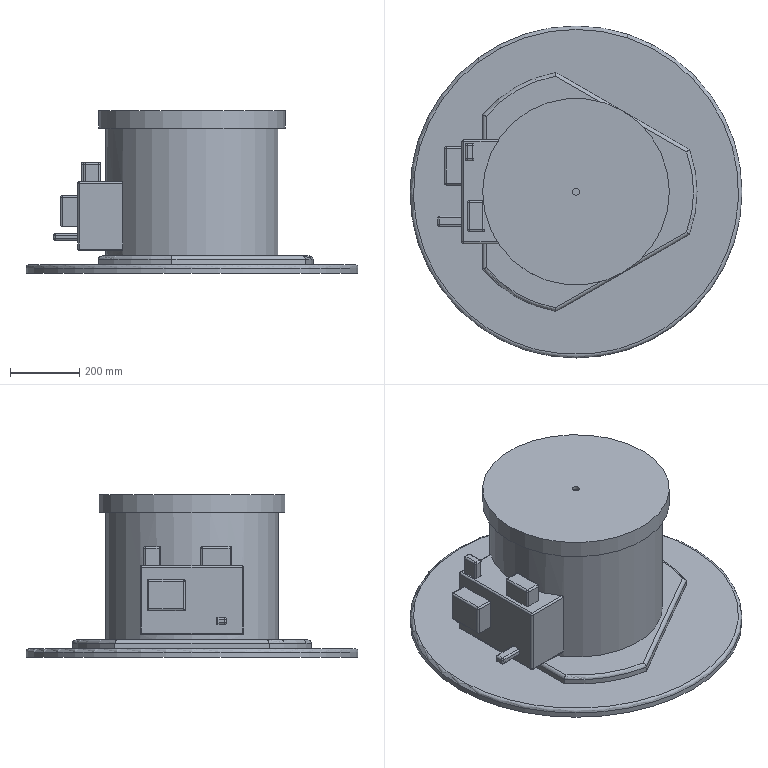Component | NX | 1_BASE | 1 solid | 106 faces | volume 116470333 mm3 | cylinder 49 | plane 34 | sphere 19 | torus 4 | commonest cylinder face diameters 10 x39 20 x4 700 x3 960 x1 500 x1 540 x1